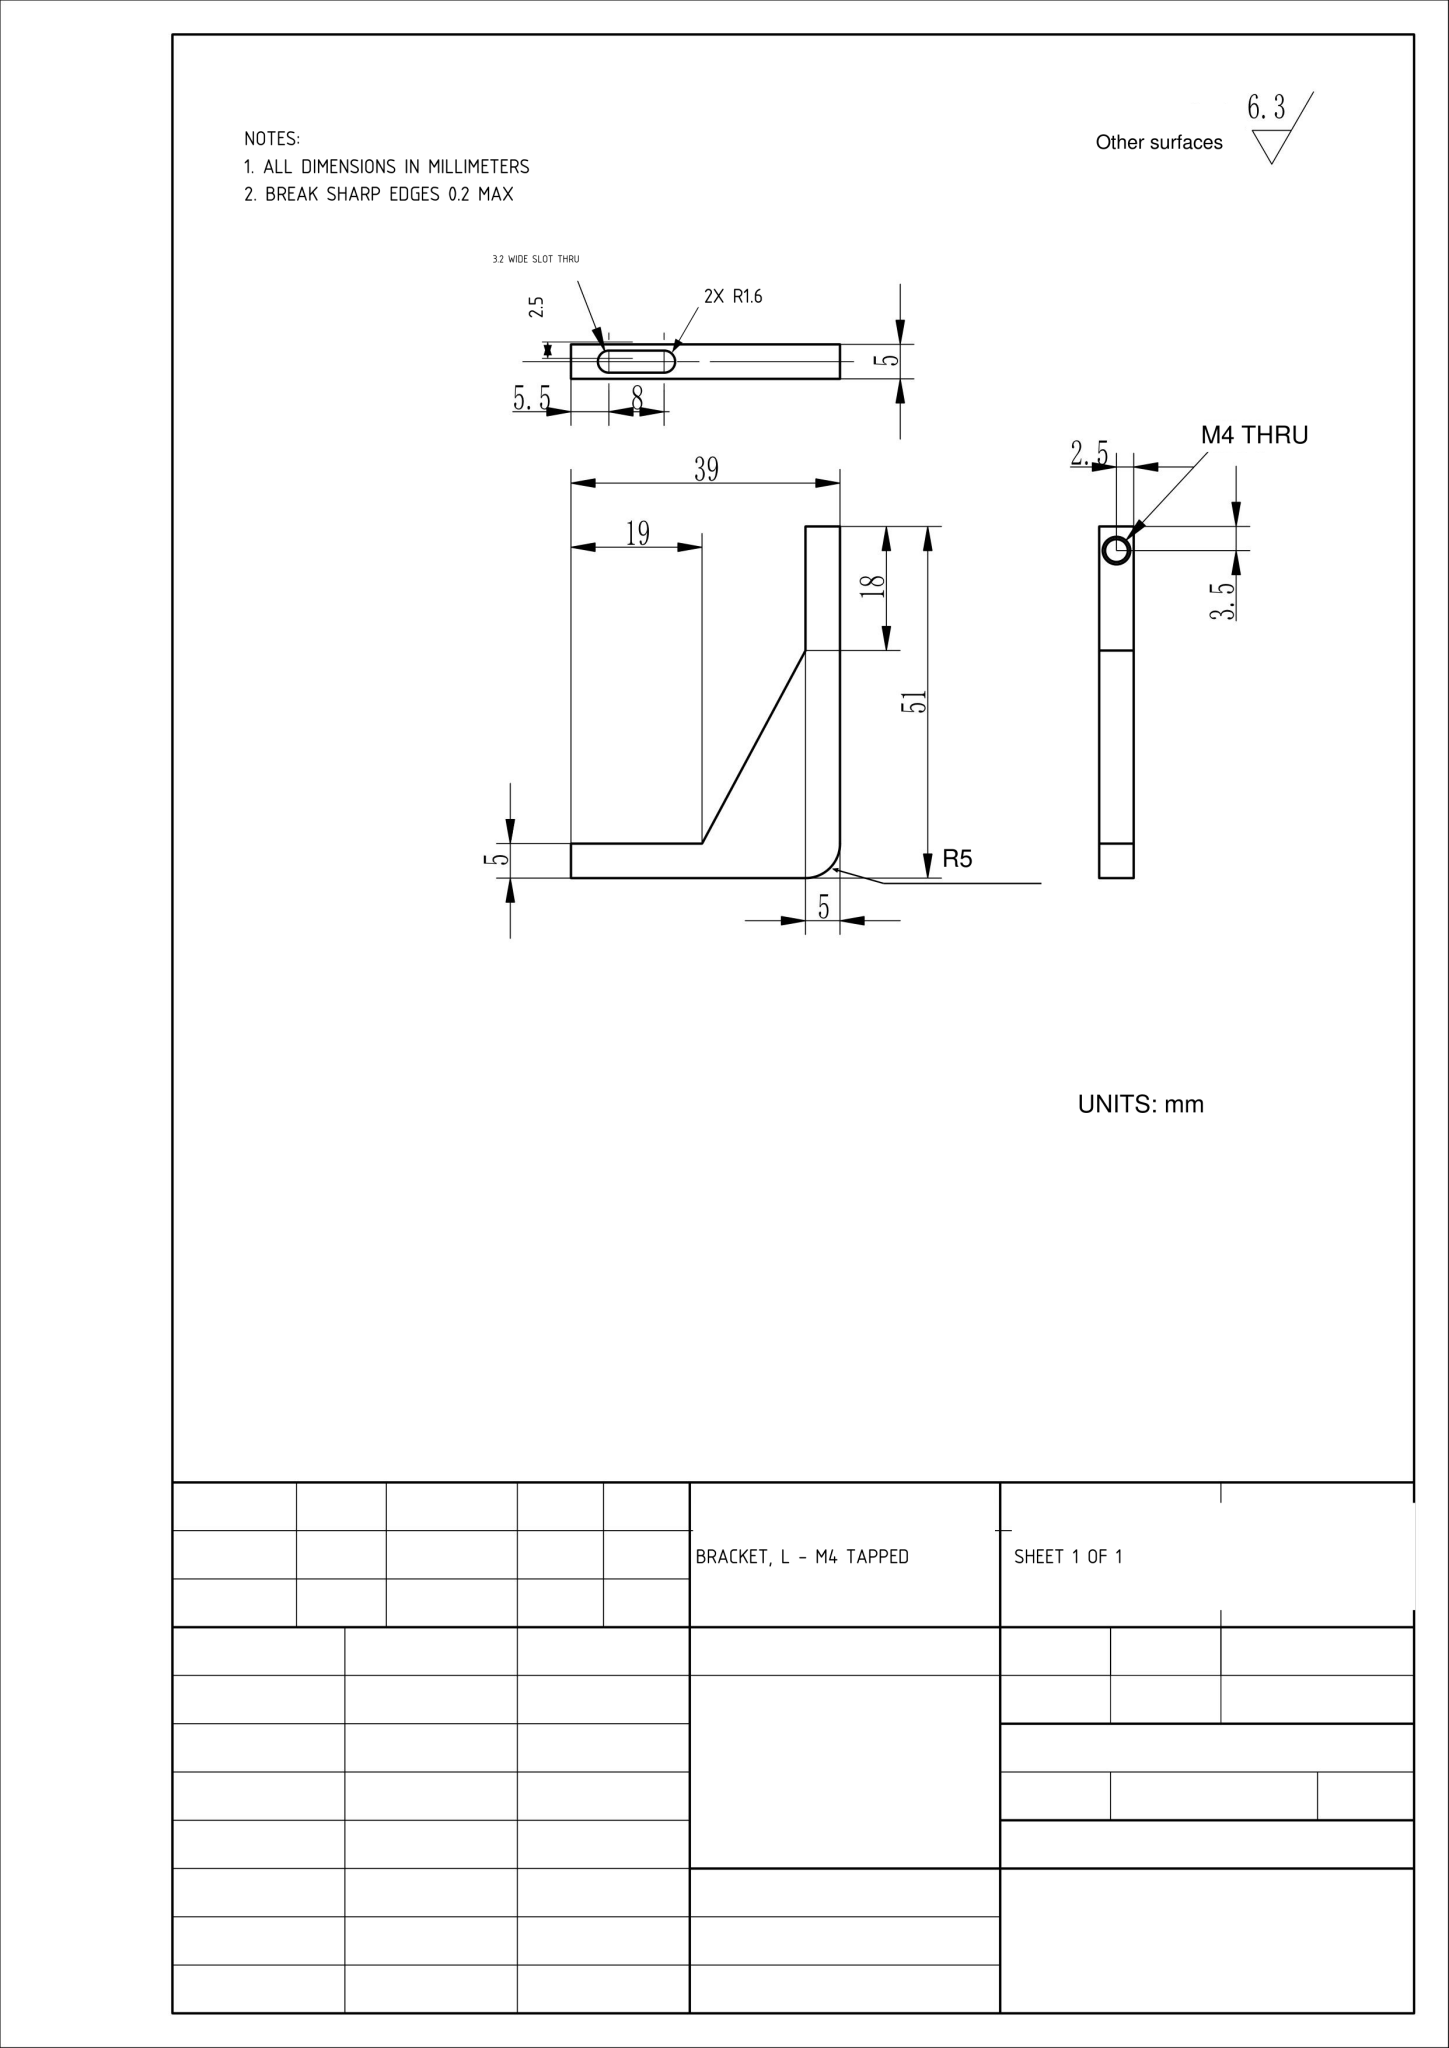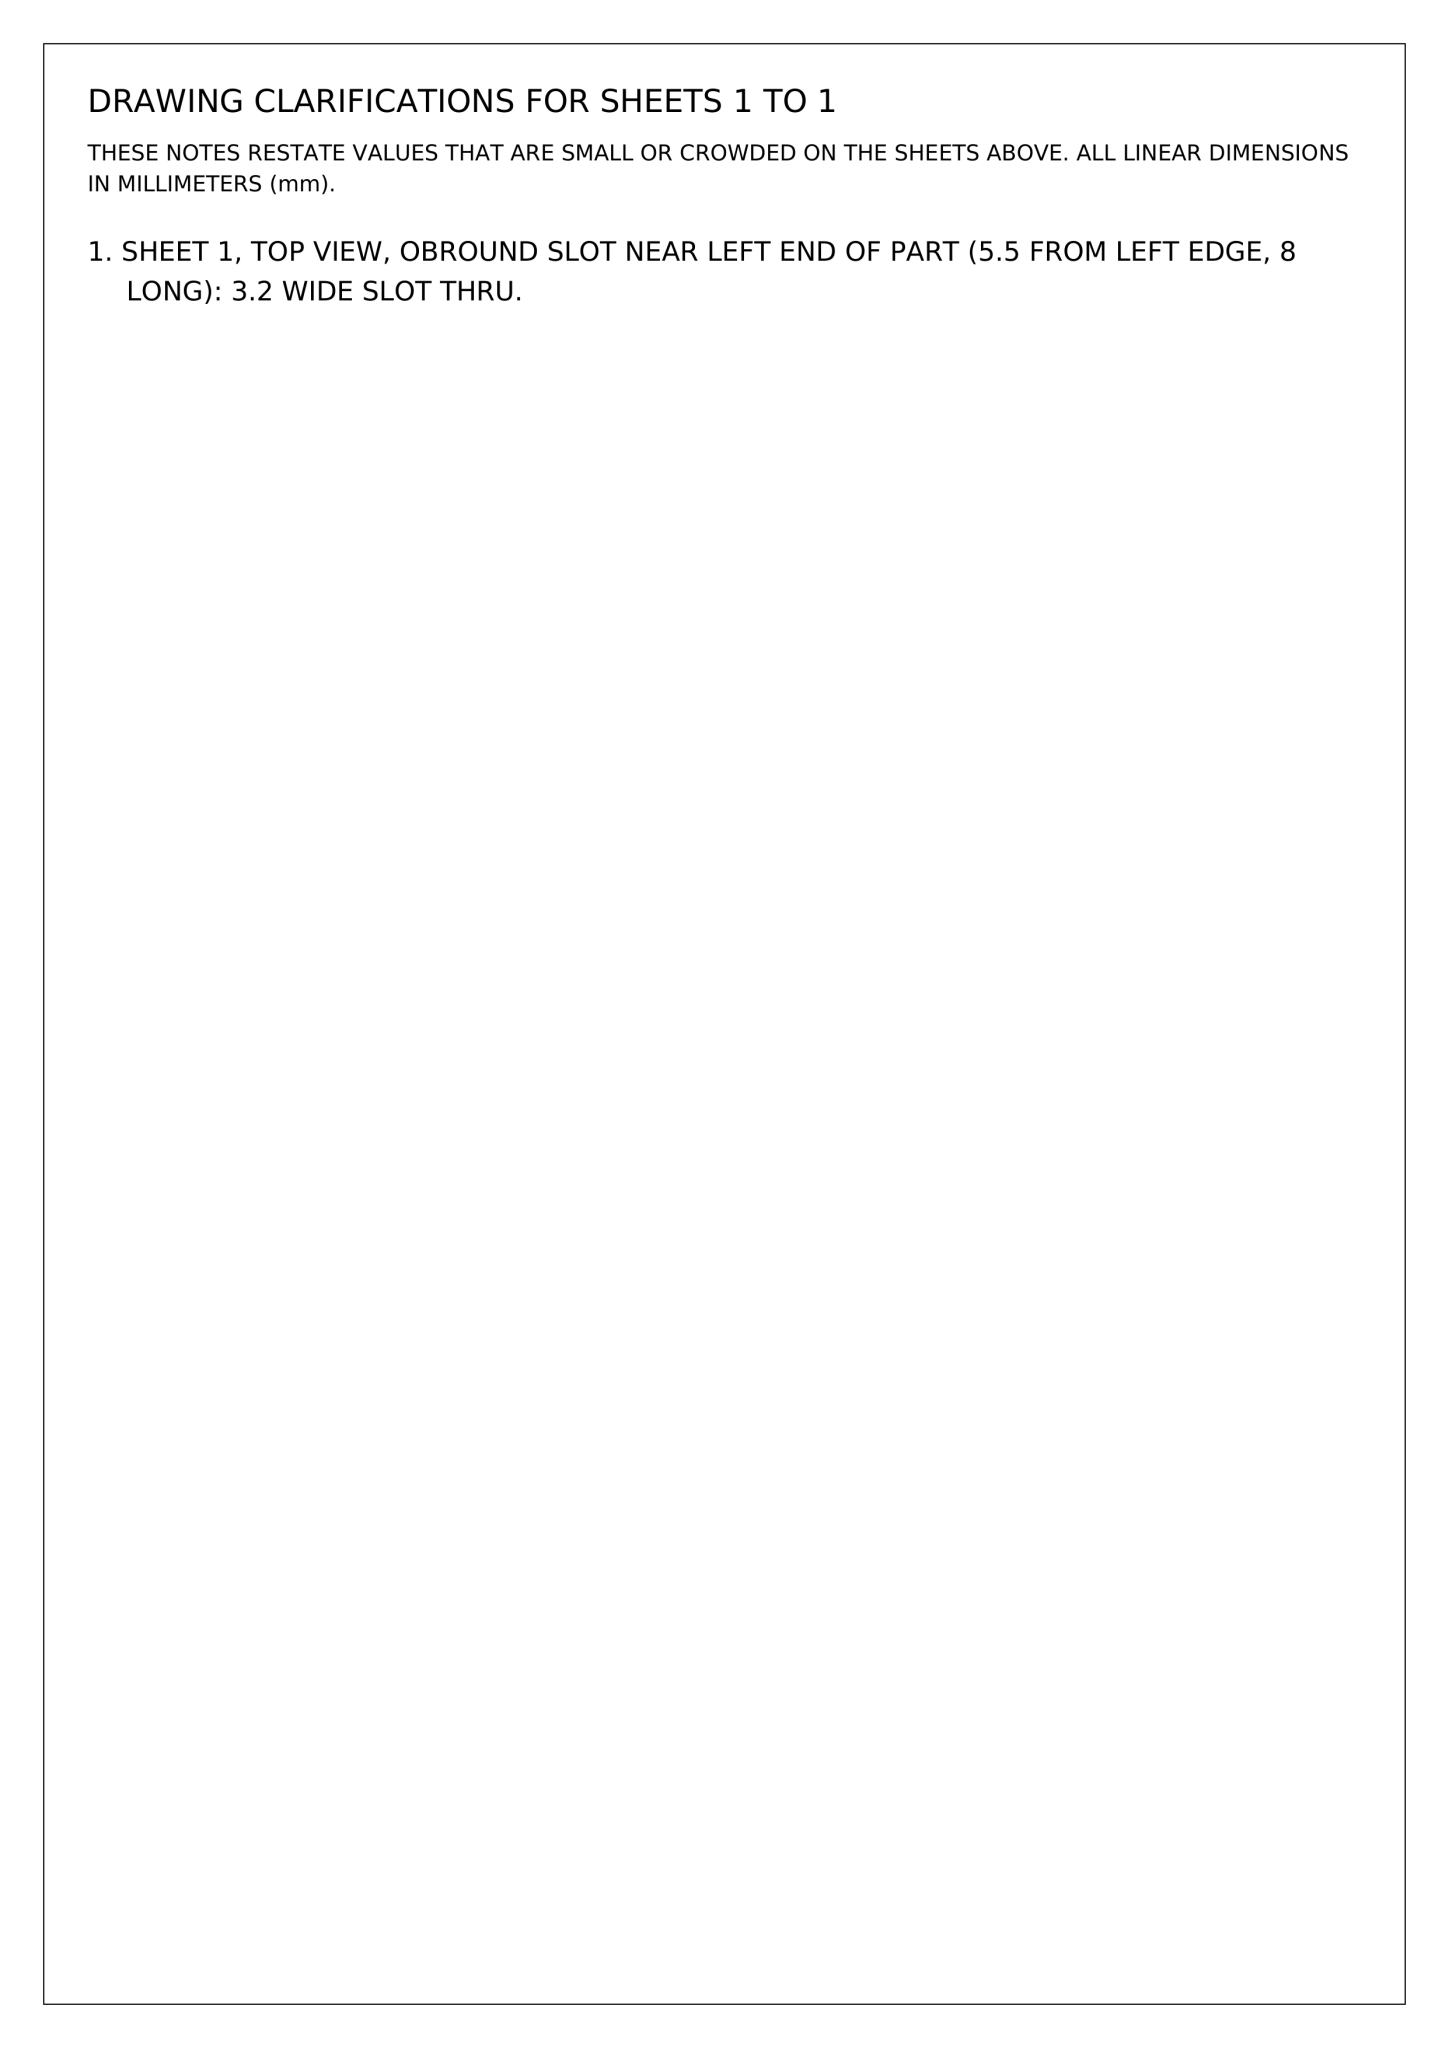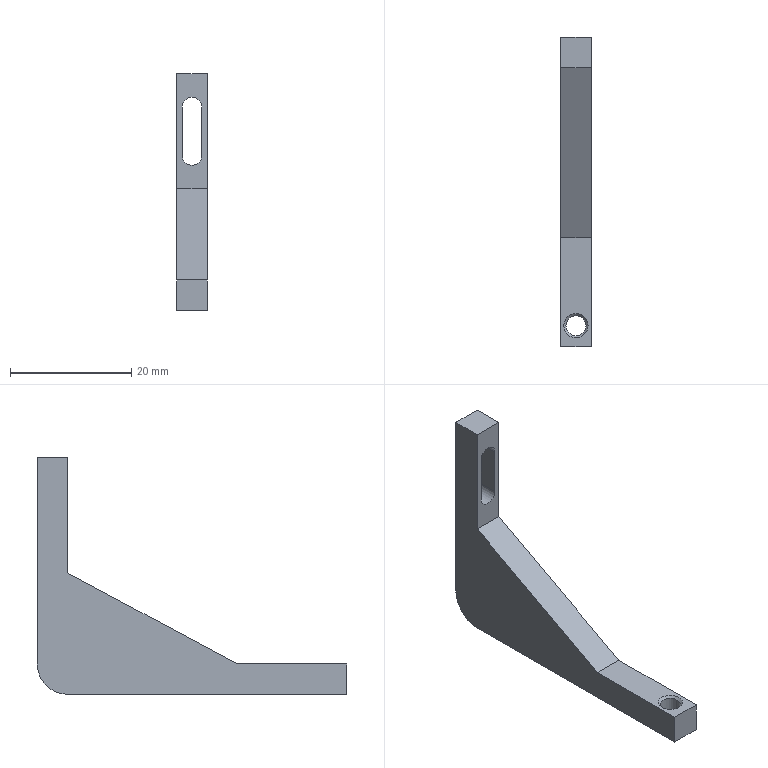Part | NX | mm | 1 solid | 17 faces | box 5 x 51 x 39 mm | volume 2936 mm3 | plane 11 | cylinder 4 | cone 2 | commonest cylinder face diameters 3.2 x2 3.3 x1 10 x1
STEP:
#1=CARTESIAN_POINT('',(0.,0.,0.));
#2=DIRECTION('',(0.,0.,1.));
#3=DIRECTION('',(1.,0.,0.));
#4=AXIS2_PLACEMENT_3D('',#1,#2,#3);
#5=(LENGTH_UNIT()NAMED_UNIT(*)SI_UNIT(.MILLI.,.METRE.));
#6=UNCERTAINTY_MEASURE_WITH_UNIT(LENGTH_MEASURE(0.00002),#5,'','');
#7=(NAMED_UNIT(*)PLANE_ANGLE_UNIT()SI_UNIT($,.RADIAN.));
#8=PLANE_ANGLE_MEASURE_WITH_UNIT(PLANE_ANGLE_MEASURE(0.01745),#7);
#9=DIMENSIONAL_EXPONENTS(0.,0.,0.,0.,0.,0.,0.);
#10=(CONVERSION_BASED_UNIT('',#8)NAMED_UNIT(#9)PLANE_ANGLE_UNIT());
#11=(NAMED_UNIT(*)SI_UNIT($,.STERADIAN.)SOLID_ANGLE_UNIT());
#12=(GEOMETRIC_REPRESENTATION_CONTEXT(3)GLOBAL_UNCERTAINTY_ASSIGNED_CONTEXT((#6))GLOBAL_UNIT_ASSIGNED_CONTEXT((#5,#10,#11))REPRESENTATION_CONTEXT('',''));
#13=SHAPE_REPRESENTATION('',(#4),#12);
#14=CARTESIAN_POINT('',(5.,46.,20.));
#15=VERTEX_POINT('',#14);
#16=CARTESIAN_POINT('',(0.,46.,20.));
#17=VERTEX_POINT('',#16);
#18=CARTESIAN_POINT('',(5.,46.,20.));
#19=DIRECTION('',(-1.,0.,0.));
#20=VECTOR('',#19,1.);
#21=LINE('',#18,#20);
#22=EDGE_CURVE('',#15,#17,#21,.T.);
#23=ORIENTED_EDGE('',*,*,#22,.F.);
#24=CARTESIAN_POINT('',(5.,46.,39.));
#25=VERTEX_POINT('',#24);
#26=CARTESIAN_POINT('',(5.,46.,39.));
#27=DIRECTION('',(0.,0.,-1.));
#28=VECTOR('',#27,1.);
#29=LINE('',#26,#28);
#30=EDGE_CURVE('',#25,#15,#29,.T.);
#31=ORIENTED_EDGE('',*,*,#30,.F.);
#32=CARTESIAN_POINT('',(0.,46.,39.));
#33=VERTEX_POINT('',#32);
#34=CARTESIAN_POINT('',(5.,46.,39.));
#35=DIRECTION('',(-1.,0.,0.));
#36=VECTOR('',#35,1.);
#37=LINE('',#34,#36);
#38=EDGE_CURVE('',#25,#33,#37,.T.);
#39=ORIENTED_EDGE('',*,*,#38,.T.);
#40=CARTESIAN_POINT('',(0.,46.,39.));
#41=DIRECTION('',(0.,0.,-1.));
#42=VECTOR('',#41,1.);
#43=LINE('',#40,#42);
#44=EDGE_CURVE('',#33,#17,#43,.T.);
#45=ORIENTED_EDGE('',*,*,#44,.T.);
#46=EDGE_LOOP('',(#23,#31,#39,#45));
#47=FACE_BOUND('',#46,.T.);
#48=CARTESIAN_POINT('',(0.9,46.,33.5));
#49=VERTEX_POINT('',#48);
#50=CARTESIAN_POINT('',(0.9,46.,25.5));
#51=VERTEX_POINT('',#50);
#52=CARTESIAN_POINT('',(0.9,46.,33.5));
#53=DIRECTION('',(0.,0.,-1.));
#54=VECTOR('',#53,1.);
#55=LINE('',#52,#54);
#56=EDGE_CURVE('',#49,#51,#55,.T.);
#57=ORIENTED_EDGE('',*,*,#56,.F.);
#58=CARTESIAN_POINT('',(4.1,46.,33.5));
#59=VERTEX_POINT('',#58);
#60=CARTESIAN_POINT('',(2.5,46.,33.5));
#61=DIRECTION('',(0.,-1.,0.));
#62=DIRECTION('',(0.,0.,-1.));
#63=AXIS2_PLACEMENT_3D('',#60,#61,#62);
#64=CIRCLE('',#63,1.6);
#65=EDGE_CURVE('',#59,#49,#64,.T.);
#66=ORIENTED_EDGE('',*,*,#65,.F.);
#67=CARTESIAN_POINT('',(4.1,46.,25.5));
#68=VERTEX_POINT('',#67);
#69=CARTESIAN_POINT('',(4.1,46.,25.5));
#70=DIRECTION('',(-0.,0.,1.));
#71=VECTOR('',#70,1.);
#72=LINE('',#69,#71);
#73=EDGE_CURVE('',#68,#59,#72,.T.);
#74=ORIENTED_EDGE('',*,*,#73,.F.);
#75=CARTESIAN_POINT('',(2.5,46.,25.5));
#76=DIRECTION('',(0.,-1.,0.));
#77=DIRECTION('',(0.,0.,-1.));
#78=AXIS2_PLACEMENT_3D('',#75,#76,#77);
#79=CIRCLE('',#78,1.6);
#80=EDGE_CURVE('',#51,#68,#79,.T.);
#81=ORIENTED_EDGE('',*,*,#80,.F.);
#82=EDGE_LOOP('',(#57,#66,#74,#81));
#83=FACE_BOUND('',#82,.T.);
#84=CARTESIAN_POINT('',(5.,46.,39.));
#85=DIRECTION('',(0.,1.,0.));
#86=DIRECTION('',(0.,-0.,1.));
#87=AXIS2_PLACEMENT_3D('',#84,#85,#86);
#88=PLANE('',#87);
#89=ADVANCED_FACE('',(#47,#83),#88,.F.);
#90=CARTESIAN_POINT('',(0.,0.,5.));
#91=VERTEX_POINT('',#90);
#92=CARTESIAN_POINT('',(0.,-0.,0.));
#93=VERTEX_POINT('',#92);
#94=CARTESIAN_POINT('',(0.,0.,5.));
#95=DIRECTION('',(0.,-0.,-1.));
#96=VECTOR('',#95,1.);
#97=LINE('',#94,#96);
#98=EDGE_CURVE('',#91,#93,#97,.T.);
#99=ORIENTED_EDGE('',*,*,#98,.T.);
#100=CARTESIAN_POINT('',(5.,-0.,0.));
#101=VERTEX_POINT('',#100);
#102=CARTESIAN_POINT('',(5.,-0.,0.));
#103=DIRECTION('',(-1.,0.,0.));
#104=VECTOR('',#103,1.);
#105=LINE('',#102,#104);
#106=EDGE_CURVE('',#101,#93,#105,.T.);
#107=ORIENTED_EDGE('',*,*,#106,.F.);
#108=CARTESIAN_POINT('',(5.,0.,5.));
#109=VERTEX_POINT('',#108);
#110=CARTESIAN_POINT('',(5.,0.,5.));
#111=DIRECTION('',(0.,-0.,-1.));
#112=VECTOR('',#111,1.);
#113=LINE('',#110,#112);
#114=EDGE_CURVE('',#109,#101,#113,.T.);
#115=ORIENTED_EDGE('',*,*,#114,.F.);
#116=CARTESIAN_POINT('',(5.,0.,5.));
#117=DIRECTION('',(-1.,0.,0.));
#118=VECTOR('',#117,1.);
#119=LINE('',#116,#118);
#120=EDGE_CURVE('',#109,#91,#119,.T.);
#121=ORIENTED_EDGE('',*,*,#120,.T.);
#122=EDGE_LOOP('',(#99,#107,#115,#121));
#123=FACE_OUTER_BOUND('',#122,.T.);
#124=CARTESIAN_POINT('',(5.,0.,5.));
#125=DIRECTION('',(0.,1.,-0.));
#126=DIRECTION('',(0.,0.,1.));
#127=AXIS2_PLACEMENT_3D('',#124,#125,#126);
#128=PLANE('',#127);
#129=ADVANCED_FACE('',(#123),#128,.F.);
#130=CARTESIAN_POINT('',(4.5,3.5,0.));
#131=VERTEX_POINT('',#130);
#132=CARTESIAN_POINT('',(2.5,3.5,0.));
#133=DIRECTION('',(0.,0.,1.));
#134=DIRECTION('',(1.,0.,0.));
#135=AXIS2_PLACEMENT_3D('',#132,#133,#134);
#136=CIRCLE('',#135,2.);
#137=EDGE_CURVE('',#131,#131,#136,.T.);
#138=ORIENTED_EDGE('',*,*,#137,.T.);
#139=EDGE_LOOP('',(#138));
#140=FACE_BOUND('',#139,.T.);
#141=CARTESIAN_POINT('',(0.,46.,0.));
#142=VERTEX_POINT('',#141);
#143=CARTESIAN_POINT('',(0.,46.,0.));
#144=DIRECTION('',(0.,1.,0.));
#145=VECTOR('',#144,1.);
#146=LINE('',#143,#145);
#147=EDGE_CURVE('',#93,#142,#146,.T.);
#148=ORIENTED_EDGE('',*,*,#147,.T.);
#149=CARTESIAN_POINT('',(5.,46.,0.));
#150=VERTEX_POINT('',#149);
#151=CARTESIAN_POINT('',(5.,46.,0.));
#152=DIRECTION('',(1.,0.,0.));
#153=VECTOR('',#152,1.);
#154=LINE('',#151,#153);
#155=EDGE_CURVE('',#142,#150,#154,.T.);
#156=ORIENTED_EDGE('',*,*,#155,.T.);
#157=CARTESIAN_POINT('',(5.,0.,0.));
#158=DIRECTION('',(0.,1.,0.));
#159=VECTOR('',#158,1.);
#160=LINE('',#157,#159);
#161=EDGE_CURVE('',#101,#150,#160,.T.);
#162=ORIENTED_EDGE('',*,*,#161,.F.);
#163=ORIENTED_EDGE('',*,*,#106,.T.);
#164=EDGE_LOOP('',(#148,#156,#162,#163));
#165=FACE_BOUND('',#164,.T.);
#166=CARTESIAN_POINT('',(5.,46.,0.));
#167=DIRECTION('',(0.,0.,1.));
#168=DIRECTION('',(1.,0.,0.));
#169=AXIS2_PLACEMENT_3D('',#166,#167,#168);
#170=PLANE('',#169);
#171=ADVANCED_FACE('',(#140,#165),#170,.F.);
#172=CARTESIAN_POINT('',(4.1,51.,33.5));
#173=VERTEX_POINT('',#172);
#174=CARTESIAN_POINT('',(0.9,51.,33.5));
#175=VERTEX_POINT('',#174);
#176=CARTESIAN_POINT('',(2.5,51.,33.5));
#177=DIRECTION('',(0.,-1.,-0.));
#178=DIRECTION('',(0.,0.,-1.));
#179=AXIS2_PLACEMENT_3D('',#176,#177,#178);
#180=CIRCLE('',#179,1.6);
#181=EDGE_CURVE('',#173,#175,#180,.T.);
#182=ORIENTED_EDGE('',*,*,#181,.T.);
#183=CARTESIAN_POINT('',(0.9,51.,25.5));
#184=VERTEX_POINT('',#183);
#185=CARTESIAN_POINT('',(0.9,51.,5.));
#186=DIRECTION('',(0.,0.,-1.));
#187=VECTOR('',#186,1.);
#188=LINE('',#185,#187);
#189=EDGE_CURVE('',#175,#184,#188,.T.);
#190=ORIENTED_EDGE('',*,*,#189,.T.);
#191=CARTESIAN_POINT('',(4.1,51.,25.5));
#192=VERTEX_POINT('',#191);
#193=CARTESIAN_POINT('',(2.5,51.,25.5));
#194=DIRECTION('',(0.,-1.,-0.));
#195=DIRECTION('',(0.,0.,-1.));
#196=AXIS2_PLACEMENT_3D('',#193,#194,#195);
#197=CIRCLE('',#196,1.6);
#198=EDGE_CURVE('',#184,#192,#197,.T.);
#199=ORIENTED_EDGE('',*,*,#198,.T.);
#200=CARTESIAN_POINT('',(4.1,51.,5.));
#201=DIRECTION('',(-0.,-0.,1.));
#202=VECTOR('',#201,1.);
#203=LINE('',#200,#202);
#204=EDGE_CURVE('',#192,#173,#203,.T.);
#205=ORIENTED_EDGE('',*,*,#204,.T.);
#206=EDGE_LOOP('',(#182,#190,#199,#205));
#207=FACE_BOUND('',#206,.T.);
#208=CARTESIAN_POINT('',(5.,51.,5.));
#209=VERTEX_POINT('',#208);
#210=CARTESIAN_POINT('',(5.,51.,39.));
#211=VERTEX_POINT('',#210);
#212=CARTESIAN_POINT('',(5.,51.,0.));
#213=DIRECTION('',(0.,0.,1.));
#214=VECTOR('',#213,1.);
#215=LINE('',#212,#214);
#216=EDGE_CURVE('',#209,#211,#215,.T.);
#217=ORIENTED_EDGE('',*,*,#216,.F.);
#218=CARTESIAN_POINT('',(0.,51.,5.));
#219=VERTEX_POINT('',#218);
#220=CARTESIAN_POINT('',(5.,51.,5.));
#221=DIRECTION('',(-1.,0.,0.));
#222=VECTOR('',#221,1.);
#223=LINE('',#220,#222);
#224=EDGE_CURVE('',#209,#219,#223,.T.);
#225=ORIENTED_EDGE('',*,*,#224,.T.);
#226=CARTESIAN_POINT('',(0.,51.,39.));
#227=VERTEX_POINT('',#226);
#228=CARTESIAN_POINT('',(0.,51.,5.));
#229=DIRECTION('',(0.,-0.,1.));
#230=VECTOR('',#229,1.);
#231=LINE('',#228,#230);
#232=EDGE_CURVE('',#219,#227,#231,.T.);
#233=ORIENTED_EDGE('',*,*,#232,.T.);
#234=CARTESIAN_POINT('',(5.,51.,39.));
#235=DIRECTION('',(-1.,0.,0.));
#236=VECTOR('',#235,1.);
#237=LINE('',#234,#236);
#238=EDGE_CURVE('',#211,#227,#237,.T.);
#239=ORIENTED_EDGE('',*,*,#238,.F.);
#240=EDGE_LOOP('',(#217,#225,#233,#239));
#241=FACE_BOUND('',#240,.T.);
#242=CARTESIAN_POINT('',(5.,51.,5.));
#243=DIRECTION('',(0.,-1.,-0.));
#244=DIRECTION('',(0.,0.,-1.));
#245=AXIS2_PLACEMENT_3D('',#242,#243,#244);
#246=PLANE('',#245);
#247=ADVANCED_FACE('',(#207,#241),#246,.F.);
#248=CARTESIAN_POINT('',(0.,51.,39.));
#249=DIRECTION('',(0.,-1.,0.));
#250=VECTOR('',#249,1.);
#251=LINE('',#248,#250);
#252=EDGE_CURVE('',#227,#33,#251,.T.);
#253=ORIENTED_EDGE('',*,*,#252,.T.);
#254=ORIENTED_EDGE('',*,*,#38,.F.);
#255=CARTESIAN_POINT('',(5.,51.,39.));
#256=DIRECTION('',(0.,-1.,0.));
#257=VECTOR('',#256,1.);
#258=LINE('',#255,#257);
#259=EDGE_CURVE('',#211,#25,#258,.T.);
#260=ORIENTED_EDGE('',*,*,#259,.F.);
#261=ORIENTED_EDGE('',*,*,#238,.T.);
#262=EDGE_LOOP('',(#253,#254,#260,#261));
#263=FACE_OUTER_BOUND('',#262,.T.);
#264=CARTESIAN_POINT('',(5.,51.,39.));
#265=DIRECTION('',(0.,0.,-1.));
#266=DIRECTION('',(-1.,0.,0.));
#267=AXIS2_PLACEMENT_3D('',#264,#265,#266);
#268=PLANE('',#267);
#269=ADVANCED_FACE('',(#263),#268,.F.);
#270=CARTESIAN_POINT('',(2.5,5.5,5.));
#271=VERTEX_POINT('',#270);
#272=CARTESIAN_POINT('',(2.5,3.5,5.));
#273=DIRECTION('',(0.,0.,-1.));
#274=DIRECTION('',(0.,1.,0.));
#275=AXIS2_PLACEMENT_3D('',#272,#273,#274);
#276=CIRCLE('',#275,2.);
#277=EDGE_CURVE('',#271,#271,#276,.T.);
#278=ORIENTED_EDGE('',*,*,#277,.T.);
#279=EDGE_LOOP('',(#278));
#280=FACE_BOUND('',#279,.T.);
#281=CARTESIAN_POINT('',(5.,18.,5.));
#282=VERTEX_POINT('',#281);
#283=CARTESIAN_POINT('',(5.,46.,5.));
#284=DIRECTION('',(0.,-1.,-0.));
#285=VECTOR('',#284,1.);
#286=LINE('',#283,#285);
#287=EDGE_CURVE('',#282,#109,#286,.T.);
#288=ORIENTED_EDGE('',*,*,#287,.F.);
#289=CARTESIAN_POINT('',(0.,18.,5.));
#290=VERTEX_POINT('',#289);
#291=CARTESIAN_POINT('',(5.,18.,5.));
#292=DIRECTION('',(-1.,0.,0.));
#293=VECTOR('',#292,1.);
#294=LINE('',#291,#293);
#295=EDGE_CURVE('',#282,#290,#294,.T.);
#296=ORIENTED_EDGE('',*,*,#295,.T.);
#297=CARTESIAN_POINT('',(0.,46.,5.));
#298=DIRECTION('',(0.,-1.,-0.));
#299=VECTOR('',#298,1.);
#300=LINE('',#297,#299);
#301=EDGE_CURVE('',#290,#91,#300,.T.);
#302=ORIENTED_EDGE('',*,*,#301,.T.);
#303=ORIENTED_EDGE('',*,*,#120,.F.);
#304=EDGE_LOOP('',(#288,#296,#302,#303));
#305=FACE_BOUND('',#304,.T.);
#306=CARTESIAN_POINT('',(5.,46.,5.));
#307=DIRECTION('',(0.,0.,-1.));
#308=DIRECTION('',(0.,1.,0.));
#309=AXIS2_PLACEMENT_3D('',#306,#307,#308);
#310=PLANE('',#309);
#311=ADVANCED_FACE('',(#280,#305),#310,.F.);
#312=ORIENTED_EDGE('',*,*,#161,.T.);
#313=CARTESIAN_POINT('',(5.,46.,5.));
#314=DIRECTION('',(1.,0.,0.));
#315=DIRECTION('',(0.,0.,-1.));
#316=AXIS2_PLACEMENT_3D('',#313,#314,#315);
#317=CIRCLE('',#316,5.);
#318=EDGE_CURVE('',#150,#209,#317,.T.);
#319=ORIENTED_EDGE('',*,*,#318,.T.);
#320=ORIENTED_EDGE('',*,*,#216,.T.);
#321=ORIENTED_EDGE('',*,*,#259,.T.);
#322=ORIENTED_EDGE('',*,*,#30,.T.);
#323=CARTESIAN_POINT('',(5.,18.,5.));
#324=DIRECTION('',(0.,0.8815,0.4722));
#325=VECTOR('',#324,1.);
#326=LINE('',#323,#325);
#327=EDGE_CURVE('',#282,#15,#326,.T.);
#328=ORIENTED_EDGE('',*,*,#327,.F.);
#329=ORIENTED_EDGE('',*,*,#287,.T.);
#330=ORIENTED_EDGE('',*,*,#114,.T.);
#331=EDGE_LOOP('',(#312,#319,#320,#321,#322,#328,#329,#330));
#332=FACE_OUTER_BOUND('',#331,.T.);
#333=CARTESIAN_POINT('',(5.,0.,0.));
#334=DIRECTION('',(1.,0.,0.));
#335=DIRECTION('',(0.,0.,-1.));
#336=AXIS2_PLACEMENT_3D('',#333,#334,#335);
#337=PLANE('',#336);
#338=ADVANCED_FACE('',(#332),#337,.T.);
#339=ORIENTED_EDGE('',*,*,#232,.F.);
#340=CARTESIAN_POINT('',(0.,46.,5.));
#341=DIRECTION('',(-1.,0.,0.));
#342=DIRECTION('',(0.,0.,-1.));
#343=AXIS2_PLACEMENT_3D('',#340,#341,#342);
#344=CIRCLE('',#343,5.);
#345=EDGE_CURVE('',#219,#142,#344,.T.);
#346=ORIENTED_EDGE('',*,*,#345,.T.);
#347=ORIENTED_EDGE('',*,*,#147,.F.);
#348=ORIENTED_EDGE('',*,*,#98,.F.);
#349=ORIENTED_EDGE('',*,*,#301,.F.);
#350=CARTESIAN_POINT('',(0.,18.,5.));
#351=DIRECTION('',(0.,0.8815,0.4722));
#352=VECTOR('',#351,1.);
#353=LINE('',#350,#352);
#354=EDGE_CURVE('',#290,#17,#353,.T.);
#355=ORIENTED_EDGE('',*,*,#354,.T.);
#356=ORIENTED_EDGE('',*,*,#44,.F.);
#357=ORIENTED_EDGE('',*,*,#252,.F.);
#358=EDGE_LOOP('',(#339,#346,#347,#348,#349,#355,#356,#357));
#359=FACE_OUTER_BOUND('',#358,.T.);
#360=CARTESIAN_POINT('',(0.,0.,0.));
#361=DIRECTION('',(1.,0.,0.));
#362=DIRECTION('',(0.,0.,-1.));
#363=AXIS2_PLACEMENT_3D('',#360,#361,#362);
#364=PLANE('',#363);
#365=ADVANCED_FACE('',(#359),#364,.F.);
#366=CARTESIAN_POINT('',(0.85,3.5,4.65));
#367=VERTEX_POINT('',#366);
#368=CARTESIAN_POINT('',(2.5,3.5,4.65));
#369=DIRECTION('',(0.,0.,1.));
#370=DIRECTION('',(-1.,0.,0.));
#371=AXIS2_PLACEMENT_3D('',#368,#369,#370);
#372=CIRCLE('',#371,1.65);
#373=EDGE_CURVE('',#367,#367,#372,.T.);
#374=ORIENTED_EDGE('',*,*,#373,.T.);
#375=EDGE_LOOP('',(#374));
#376=FACE_BOUND('',#375,.T.);
#377=CARTESIAN_POINT('',(4.15,3.5,0.35));
#378=VERTEX_POINT('',#377);
#379=CARTESIAN_POINT('',(2.5,3.5,0.35));
#380=DIRECTION('',(0.,0.,-1.));
#381=DIRECTION('',(1.,0.,0.));
#382=AXIS2_PLACEMENT_3D('',#379,#380,#381);
#383=CIRCLE('',#382,1.65);
#384=EDGE_CURVE('',#378,#378,#383,.T.);
#385=ORIENTED_EDGE('',*,*,#384,.T.);
#386=EDGE_LOOP('',(#385));
#387=FACE_BOUND('',#386,.T.);
#388=CARTESIAN_POINT('',(2.5,3.5,0.));
#389=DIRECTION('',(0.,0.,1.));
#390=DIRECTION('',(1.,0.,0.));
#391=AXIS2_PLACEMENT_3D('',#388,#389,#390);
#392=CYLINDRICAL_SURFACE('',#391,1.65);
#393=ADVANCED_FACE('',(#376,#387),#392,.F.);
#394=ORIENTED_EDGE('',*,*,#384,.F.);
#395=EDGE_LOOP('',(#394));
#396=FACE_BOUND('',#395,.T.);
#397=ORIENTED_EDGE('',*,*,#137,.F.);
#398=EDGE_LOOP('',(#397));
#399=FACE_BOUND('',#398,.T.);
#400=CARTESIAN_POINT('',(2.5,3.5,0.));
#401=DIRECTION('',(0.,0.,-1.));
#402=DIRECTION('',(-1.,0.,0.));
#403=AXIS2_PLACEMENT_3D('',#400,#401,#402);
#404=CONICAL_SURFACE('',#403,2.,45.);
#405=ADVANCED_FACE('',(#396,#399),#404,.F.);
#406=ORIENTED_EDGE('',*,*,#373,.F.);
#407=EDGE_LOOP('',(#406));
#408=FACE_BOUND('',#407,.T.);
#409=ORIENTED_EDGE('',*,*,#277,.F.);
#410=EDGE_LOOP('',(#409));
#411=FACE_BOUND('',#410,.T.);
#412=CARTESIAN_POINT('',(2.5,3.5,5.));
#413=DIRECTION('',(0.,0.,1.));
#414=DIRECTION('',(1.,0.,0.));
#415=AXIS2_PLACEMENT_3D('',#412,#413,#414);
#416=CONICAL_SURFACE('',#415,2.,45.);
#417=ADVANCED_FACE('',(#408,#411),#416,.F.);
#418=ORIENTED_EDGE('',*,*,#354,.F.);
#419=ORIENTED_EDGE('',*,*,#295,.F.);
#420=ORIENTED_EDGE('',*,*,#327,.T.);
#421=ORIENTED_EDGE('',*,*,#22,.T.);
#422=EDGE_LOOP('',(#418,#419,#420,#421));
#423=FACE_OUTER_BOUND('',#422,.T.);
#424=CARTESIAN_POINT('',(5.,18.,5.));
#425=DIRECTION('',(0.,-0.4722,0.8815));
#426=DIRECTION('',(0.,-0.8815,-0.4722));
#427=AXIS2_PLACEMENT_3D('',#424,#425,#426);
#428=PLANE('',#427);
#429=ADVANCED_FACE('',(#423),#428,.T.);
#430=CARTESIAN_POINT('',(0.9,70.,33.5));
#431=DIRECTION('',(0.,1.,0.));
#432=VECTOR('',#431,1.);
#433=LINE('',#430,#432);
#434=EDGE_CURVE('',#49,#175,#433,.T.);
#435=ORIENTED_EDGE('',*,*,#434,.F.);
#436=ORIENTED_EDGE('',*,*,#56,.T.);
#437=CARTESIAN_POINT('',(0.9,70.,25.5));
#438=DIRECTION('',(0.,1.,0.));
#439=VECTOR('',#438,1.);
#440=LINE('',#437,#439);
#441=EDGE_CURVE('',#51,#184,#440,.T.);
#442=ORIENTED_EDGE('',*,*,#441,.T.);
#443=ORIENTED_EDGE('',*,*,#189,.F.);
#444=EDGE_LOOP('',(#435,#436,#442,#443));
#445=FACE_OUTER_BOUND('',#444,.T.);
#446=CARTESIAN_POINT('',(0.9,70.,33.5));
#447=DIRECTION('',(-1.,0.,-0.));
#448=DIRECTION('',(-0.,0.,1.));
#449=AXIS2_PLACEMENT_3D('',#446,#447,#448);
#450=PLANE('',#449);
#451=ADVANCED_FACE('',(#445),#450,.F.);
#452=ORIENTED_EDGE('',*,*,#441,.F.);
#453=ORIENTED_EDGE('',*,*,#80,.T.);
#454=CARTESIAN_POINT('',(4.1,70.,25.5));
#455=DIRECTION('',(0.,1.,0.));
#456=VECTOR('',#455,1.);
#457=LINE('',#454,#456);
#458=EDGE_CURVE('',#68,#192,#457,.T.);
#459=ORIENTED_EDGE('',*,*,#458,.T.);
#460=ORIENTED_EDGE('',*,*,#198,.F.);
#461=EDGE_LOOP('',(#452,#453,#459,#460));
#462=FACE_OUTER_BOUND('',#461,.T.);
#463=CARTESIAN_POINT('',(2.5,70.,25.5));
#464=DIRECTION('',(0.,-1.,0.));
#465=DIRECTION('',(0.,0.,-1.));
#466=AXIS2_PLACEMENT_3D('',#463,#464,#465);
#467=CYLINDRICAL_SURFACE('',#466,1.6);
#468=ADVANCED_FACE('',(#462),#467,.F.);
#469=ORIENTED_EDGE('',*,*,#458,.F.);
#470=ORIENTED_EDGE('',*,*,#73,.T.);
#471=CARTESIAN_POINT('',(4.1,70.,33.5));
#472=DIRECTION('',(0.,1.,0.));
#473=VECTOR('',#472,1.);
#474=LINE('',#471,#473);
#475=EDGE_CURVE('',#59,#173,#474,.T.);
#476=ORIENTED_EDGE('',*,*,#475,.T.);
#477=ORIENTED_EDGE('',*,*,#204,.F.);
#478=EDGE_LOOP('',(#469,#470,#476,#477));
#479=FACE_OUTER_BOUND('',#478,.T.);
#480=CARTESIAN_POINT('',(4.1,70.,25.5));
#481=DIRECTION('',(1.,0.,0.));
#482=DIRECTION('',(0.,0.,-1.));
#483=AXIS2_PLACEMENT_3D('',#480,#481,#482);
#484=PLANE('',#483);
#485=ADVANCED_FACE('',(#479),#484,.F.);
#486=ORIENTED_EDGE('',*,*,#475,.F.);
#487=ORIENTED_EDGE('',*,*,#65,.T.);
#488=ORIENTED_EDGE('',*,*,#434,.T.);
#489=ORIENTED_EDGE('',*,*,#181,.F.);
#490=EDGE_LOOP('',(#486,#487,#488,#489));
#491=FACE_OUTER_BOUND('',#490,.T.);
#492=CARTESIAN_POINT('',(2.5,70.,33.5));
#493=DIRECTION('',(0.,-1.,0.));
#494=DIRECTION('',(0.,0.,-1.));
#495=AXIS2_PLACEMENT_3D('',#492,#493,#494);
#496=CYLINDRICAL_SURFACE('',#495,1.6);
#497=ADVANCED_FACE('',(#491),#496,.F.);
#498=ORIENTED_EDGE('',*,*,#318,.F.);
#499=ORIENTED_EDGE('',*,*,#155,.F.);
#500=ORIENTED_EDGE('',*,*,#345,.F.);
#501=ORIENTED_EDGE('',*,*,#224,.F.);
#502=EDGE_LOOP('',(#498,#499,#500,#501));
#503=FACE_OUTER_BOUND('',#502,.T.);
#504=CARTESIAN_POINT('',(5.,46.,5.));
#505=DIRECTION('',(-1.,0.,0.));
#506=DIRECTION('',(0.,0.,1.));
#507=AXIS2_PLACEMENT_3D('',#504,#505,#506);
#508=CYLINDRICAL_SURFACE('',#507,5.);
#509=ADVANCED_FACE('',(#503),#508,.T.);
#510=CLOSED_SHELL('',(#89,#129,#171,#247,#269,#311,#338,#365,#393,#405,#417,#429,#451,#468,#485,#497,#509));
#511=MANIFOLD_SOLID_BREP('',#510);
#512=ADVANCED_BREP_SHAPE_REPRESENTATION('',(#511),#12);
#513=SHAPE_REPRESENTATION_RELATIONSHIP('','',#13,#512);
#514=PRESENTATION_LAYER_ASSIGNMENT('','',(#511));
#515=COLOUR_RGB('',1.,0.6,0.);
#516=FILL_AREA_STYLE_COLOUR('',#515);
#517=FILL_AREA_STYLE('',(#516));
#518=SURFACE_STYLE_FILL_AREA(#517);
#519=SURFACE_SIDE_STYLE('',(#518));
#520=SURFACE_STYLE_USAGE(.BOTH.,#519);
#521=PRESENTATION_STYLE_ASSIGNMENT((#520));
#522=STYLED_ITEM('',(#521),#511);
#523=MECHANICAL_DESIGN_GEOMETRIC_PRESENTATION_REPRESENTATION('',(#522),#12);